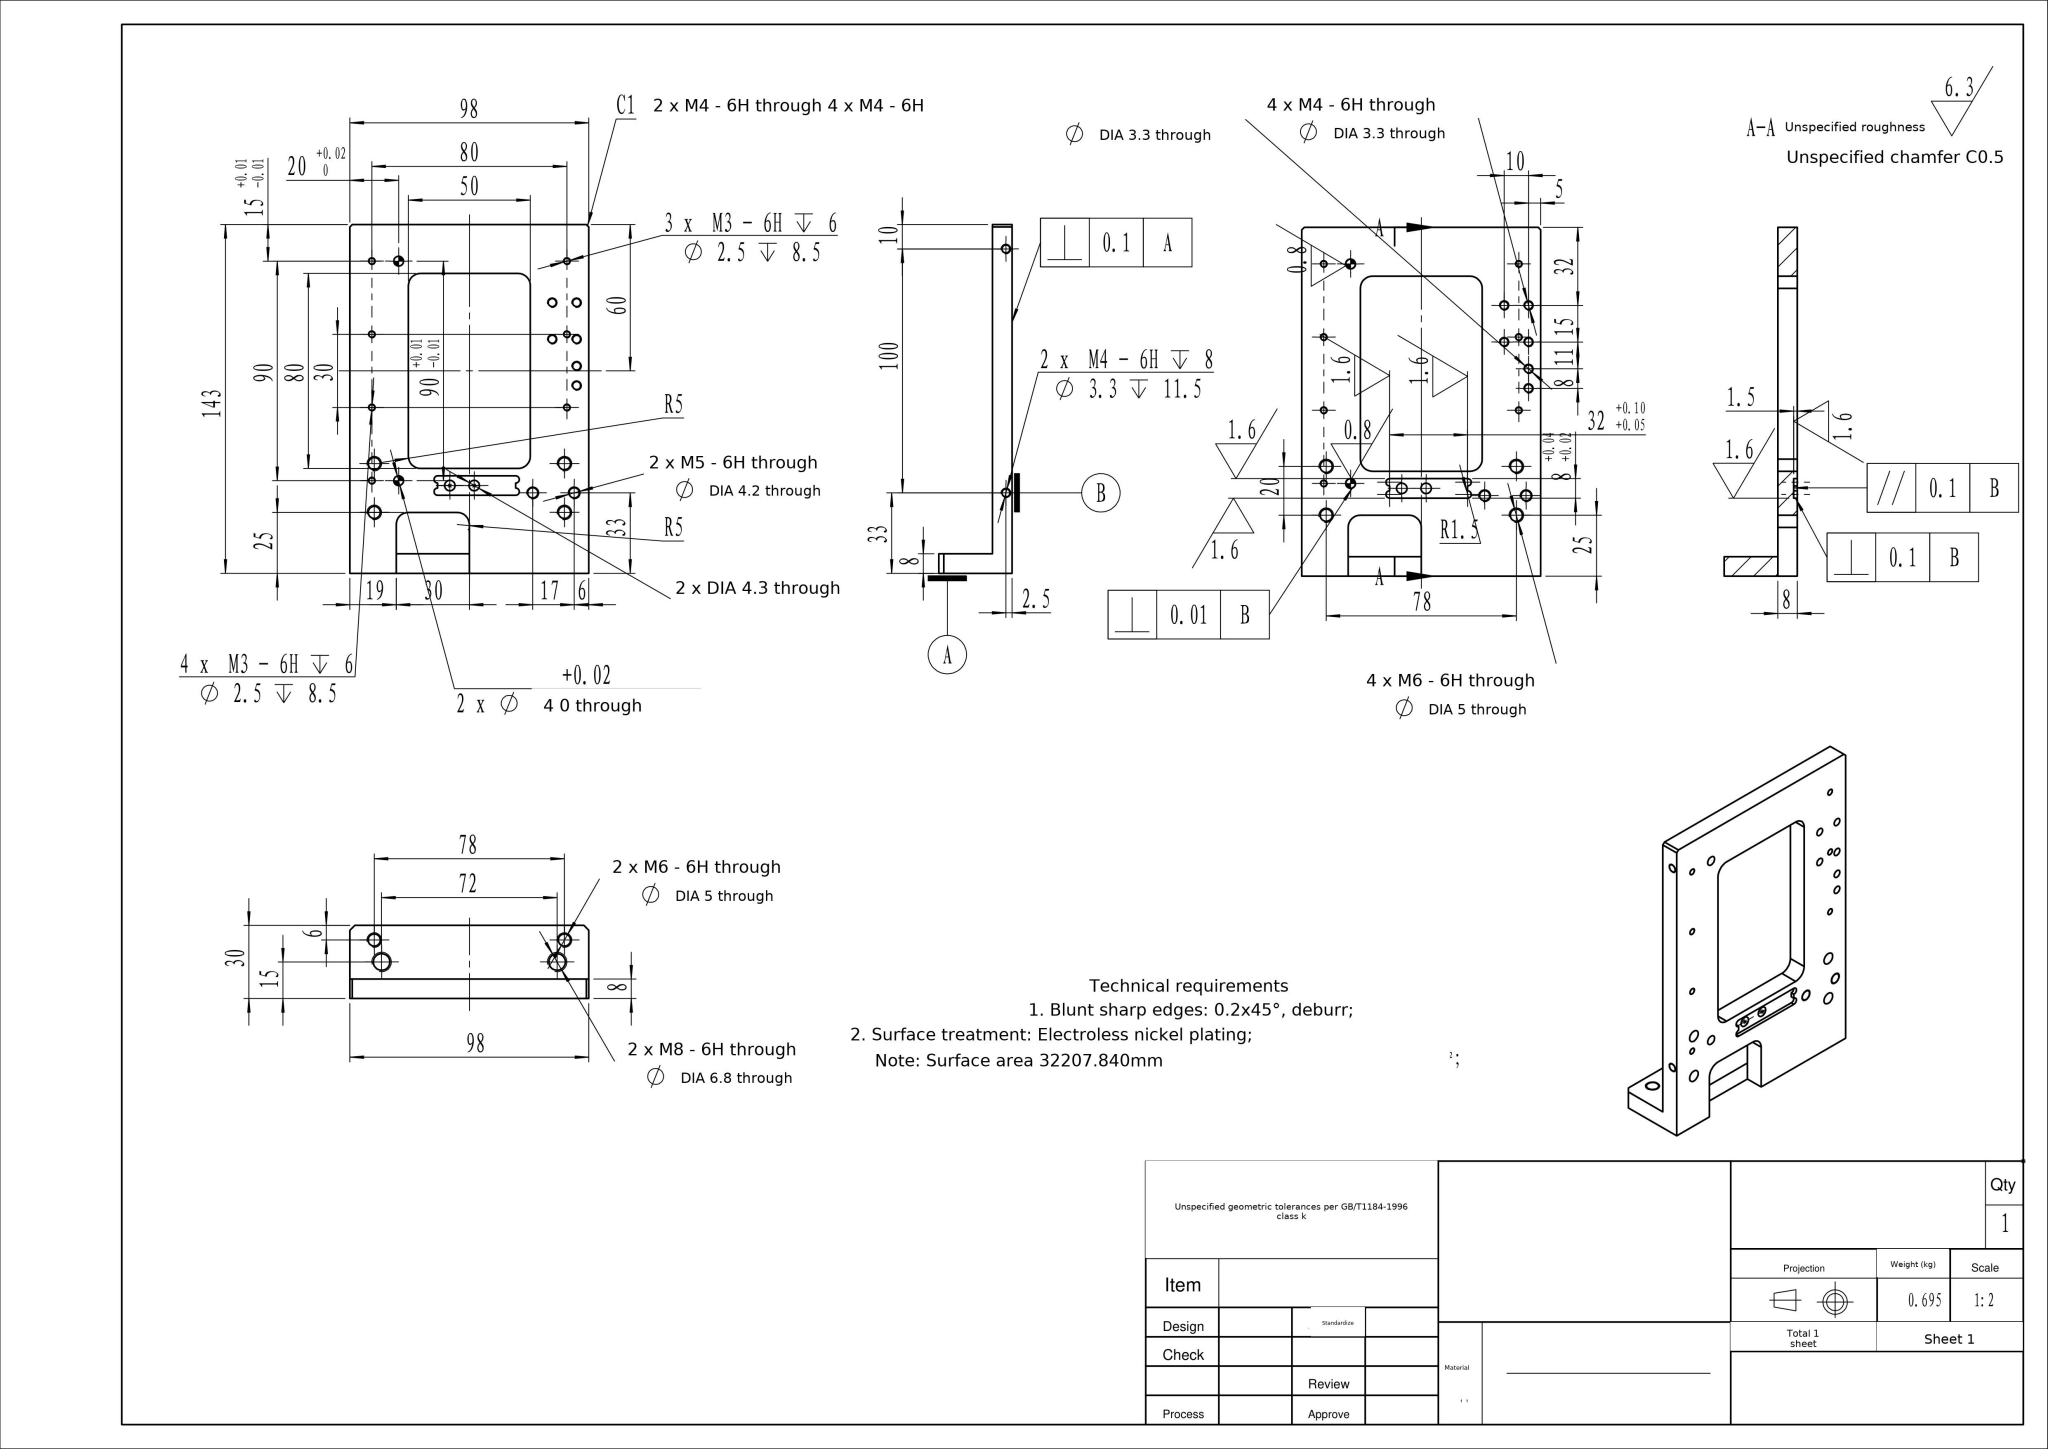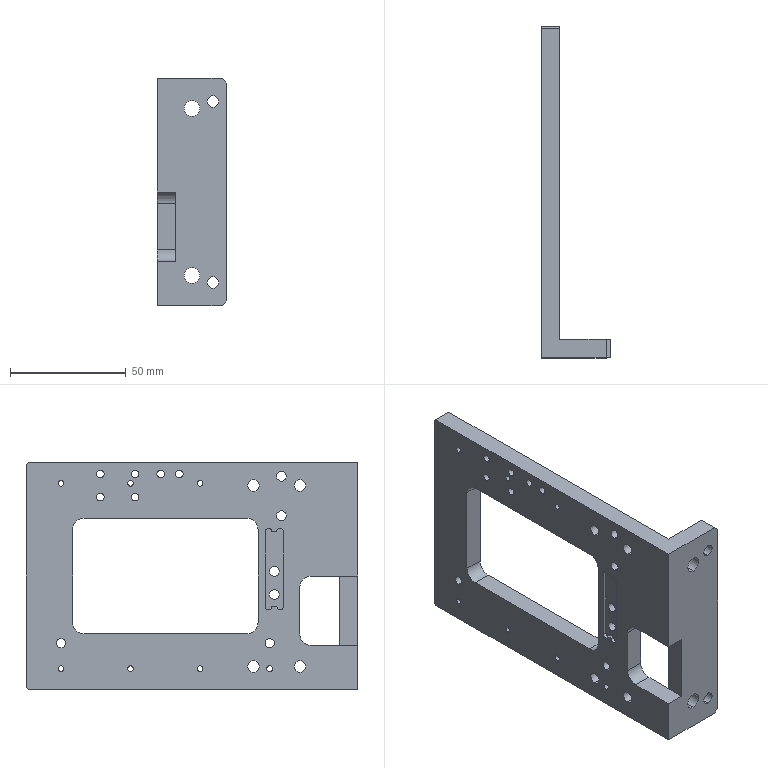Part | SolidWorks | mm | 1 solid | 99 faces | box 30 x 143 x 98 mm | volume 88149 mm3 | cylinder 70 | plane 25 | cone 4 | commonest cylinder face diameters 3.3 x16 2.5 x14 5 x12 3 x6 10 x6 4.3 x4 4 x4 4.2 x4
build123d program:
from build123d import *

# Parameters (mm, degrees)
BOSS_EXTRUDE1_DEPTH        = 98
CHAMFER1_SIZE              = 2
M8_TAPPED_HOLE1_D          = 6.8
SKETCH5_W                  = 50
SKETCH5_H                  = 80
CUT_EXTRUDE1_DEPTH         = 176.935
FILLET1_R                  = 5
SKETCH6_W                  = 30
SKETCH6_H                  = 25
CUT_EXTRUDE2_DEPTH         = 8
FILLET2_R                  = 5
M5_TAPPED_HOLE1_D          = 4.2
FILLET4_R                  = 5
LPATTERN1_COUNT            = 4
LPATTERN1_PITCH            = 30
LPATTERN2_COUNT            = 3
LPATTERN2_PITCH            = 30
F_4_0_4_DIAMETER_HOLE1_D   = 4
M4_TAPPED_HOLE1_D          = 3.3
M4_TAPPED_HOLE1_DEPTH      = 11.5
M4_TAPPED_HOLE1_TIP        = 0.9914
CHAMFER2_SIZE              = 1
SKETCH22_R                 = 1.5
SKETCH22_W                 = 32
SKETCH22_H                 = 8
CUT_EXTRUDE3_DEPTH         = 1.5
F_4_3_4_3_DIAMETER_HOLE1_D = 4.3
M4_TAPPED_HOLE2_D          = 3.3
M4_TAPPED_HOLE3_D          = 3.3
M6_TAPPED_HOLE1_D          = 5
M6_TAPPED_HOLE2_D          = 5


with BuildPart() as part:
    # Sketch1 → Boss-Extrude1 (new body)
    with BuildSketch(Plane.XY):
        Polygon((0, 0), (0, 143), (8, 143), (8, 8), (30, 8), (30, 0), align=None)
    extrude(amount=BOSS_EXTRUDE1_DEPTH)

    # Chamfer1
    chamfer1_edges = [part.edges().sort_by_distance(p)[0] for p in [
        (30, 4, 98),
        (30, 4, 0),
    ]]
    chamfer(chamfer1_edges, length=CHAMFER1_SIZE)

    # M8 Tapped Hole1 (through all)
    with Locations(Plane(origin=(0, 0, 0), x_dir=(-1, 0, 0), z_dir=(0, -1, 0))):
        with Locations((-15, -85), (-15, -13)):
            Hole(M8_TAPPED_HOLE1_D / 2)

    # Sketch5 → Cut-Extrude1 (cut, through all)
    with BuildSketch(Plane.ZY):
        with Locations((49, 83)):
            Rectangle(SKETCH5_W, SKETCH5_H)
    extrude(amount=-CUT_EXTRUDE1_DEPTH, mode=Mode.SUBTRACT)

    # Fillet1
    fillet1_edges = [part.edges().sort_by_distance(p)[0] for p in [
        (4, 123, 74),
        (4, 43, 74),
        (4, 43, 24),
        (4, 123, 24),
    ]]
    fillet(fillet1_edges, radius=FILLET1_R)

    # Sketch6 → Cut-Extrude2 (cut)
    with BuildSketch(Plane.ZY):
        with Locations((34, 12.5)):
            Rectangle(SKETCH6_W, SKETCH6_H)
    extrude(amount=-CUT_EXTRUDE2_DEPTH, mode=Mode.SUBTRACT)

    # Fillet2
    fillet2_edges = [part.edges().sort_by_distance(p)[0] for p in [
        (4, 25, 19),
    ]]
    fillet(fillet2_edges, radius=FILLET2_R)

    # M5 Tapped Hole1 (through all)
    with Locations(Plane.ZY):
        with Locations((75, 33), (92, 33)):
            Hole(M5_TAPPED_HOLE1_D / 2)

    # Fillet4
    fillet4_edges = [part.edges().sort_by_distance(p)[0] for p in [
        (4, 25, 49),
    ]]
    fillet(fillet4_edges, radius=FILLET4_R)

    # Sketch11 → M3 Tapped Hole1 (revolve, cut)
    with BuildSketch(Plane(origin=(0, 128, 9), x_dir=(0, 0, 1), z_dir=(0, 1, 0))):
        Polygon((0, 0), (0, 9.251), (1.25, 8.5), (1.25, 0), align=None)
    m3_tapped_hole1 = revolve(axis=Axis((-6.35, 128, 9), (1, 0, 0)), mode=Mode.SUBTRACT)

    # LPattern1: M3 Tapped Hole1 ×4
    with Locations(*[(0, -i * LPATTERN1_PITCH, 0) for i in range(1, LPATTERN1_COUNT)]):
        add(m3_tapped_hole1, mode=Mode.SUBTRACT)

    # Sketch14 → M3 Tapped Hole2 (revolve, cut)
    with BuildSketch(Plane(origin=(0, 128, 89), x_dir=(0, 0, 1), z_dir=(0, 1, 0))):
        Polygon((0, 0), (0, 9.251), (1.25, 8.5), (1.25, 0), align=None)
    m3_tapped_hole2 = revolve(axis=Axis((-6.35, 128, 89), (1, 0, 0)), mode=Mode.SUBTRACT)

    # LPattern2: M3 Tapped Hole2 ×3
    with Locations(*[(0, -i * LPATTERN2_PITCH, 0) for i in range(1, LPATTERN2_COUNT)]):
        add(m3_tapped_hole2, mode=Mode.SUBTRACT)

    # 4.0 _4_ Diameter Hole1 (through all)
    with Locations(Plane.ZY):
        with Locations((20, 128), (20, 38)):
            Hole(F_4_0_4_DIAMETER_HOLE1_D / 2)

    # M4 Tapped Hole1
    with Locations(Plane(origin=(0, 0, 0), x_dir=(-1, 0, 0), z_dir=(0, 0, -1))):
        with Locations((-2.5, 133), (-2.5, 33)):
            Hole(M4_TAPPED_HOLE1_D / 2, depth=M4_TAPPED_HOLE1_DEPTH)
            with Locations((0, 0, -(M4_TAPPED_HOLE1_DEPTH + M4_TAPPED_HOLE1_TIP / 2))):  # 118° drill point
                Cone(0, M4_TAPPED_HOLE1_D / 2, M4_TAPPED_HOLE1_TIP, mode=Mode.SUBTRACT)

    # Chamfer2
    chamfer2_edges = [part.edges().sort_by_distance(p)[0] for p in [
        (4, 143, 98),
        (4, 143, 0),
    ]]
    chamfer(chamfer2_edges, length=CHAMFER2_SIZE)

    # Sketch22 → Cut-Extrude3 (cut)
    with BuildSketch(Plane.ZY):
        with Locations((36, 38.5)):
            Circle(SKETCH22_R)
        with Locations((36, 33.5)):
            Circle(SKETCH22_R)
        with Locations((68, 38.5)):
            Circle(SKETCH22_R)
        with Locations((68, 33.5)):
            Circle(SKETCH22_R)
        with Locations((52, 36)):
            Rectangle(SKETCH22_W, SKETCH22_H)
    extrude(amount=-CUT_EXTRUDE3_DEPTH, mode=Mode.SUBTRACT)

    # 4.3 _4.3_ Diameter Hole1 (through all)
    with Locations(Plane.ZY.offset(-1.5)):
        with Locations((41, 36), (51, 36)):
            Hole(F_4_3_4_3_DIAMETER_HOLE1_D / 2)

    # M4 Tapped Hole2 (through all)
    with Locations(Plane(origin=(8, 0, 0), x_dir=(0, 0, -1), z_dir=(1, 0, 0))):
        with Locations((-93, 111), (-83, 111), (-93, 96), (-83, 96)):
            Hole(M4_TAPPED_HOLE2_D / 2)

    # M4 Tapped Hole3 (through all)
    with Locations(Plane(origin=(8, 0, 0), x_dir=(0, 0, -1), z_dir=(1, 0, 0))):
        with Locations((-93, 85), (-93, 77)):
            Hole(M4_TAPPED_HOLE3_D / 2)

    # M6 Tapped Hole1 (through all)
    with Locations(Plane(origin=(8, 0, 0), x_dir=(0, 0, -1), z_dir=(1, 0, 0))):
        with Locations((-88, 45), (-88, 25), (-10, 45), (-10, 25)):
            Hole(M6_TAPPED_HOLE1_D / 2)

    # M6 Tapped Hole2 (through all)
    with Locations(Plane(origin=(0, 8, 0), x_dir=(1, 0, 0), z_dir=(0, 1, 0))):
        with Locations((24, -88), (24, -10)):
            Hole(M6_TAPPED_HOLE2_D / 2)


solid = part.part